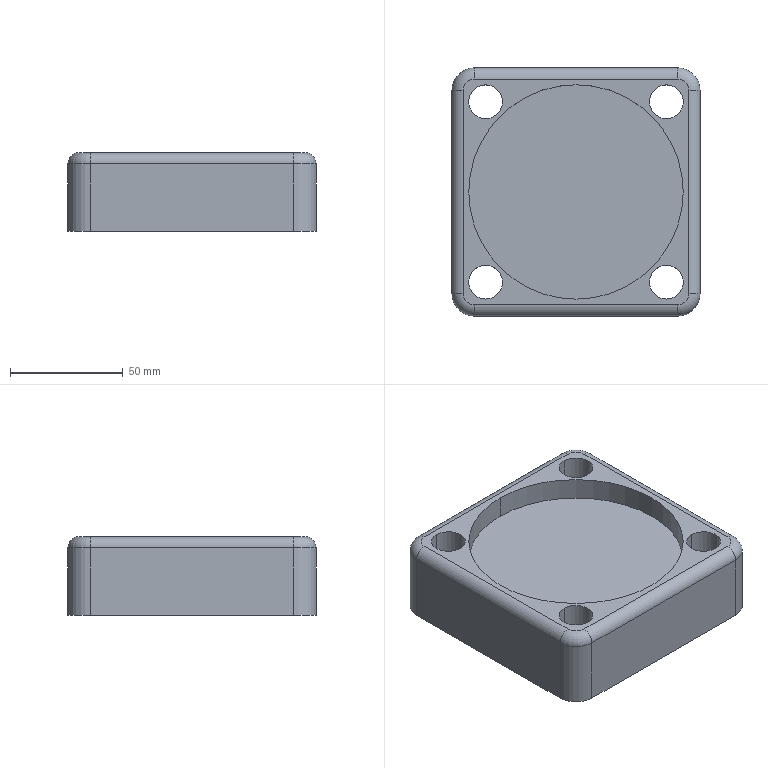Component | SolidWorks | MountingBracket-1 | 1 solid | 29 faces | box 110 x 110 x 35 mm | volume 322642 mm3 | cylinder 18 | plane 7 | torus 4 | commonest cylinder face diameters 15 x8 20 x4 10 x4 95 x2 | material 1023 Carbon Steel Plate (SS)
build123d program:
from build123d import *

# Parameters (mm, degrees)
SKETCH1_W           = 110
SKETCH1_H           = 110
BOSS_EXTRUDE1_DEPTH = 17.5
SKETCH2_R           = 47.5
CUT_EXTRUDE1_DEPTH  = 10
SKETCH3_R           = 7.5
CUT_EXTRUDE2_DEPTH  = 86.294
FILLET1_R           = 10
FILLET2_R           = 5


with BuildPart() as part:
    # Sketch1 → Boss-Extrude1 (new, symmetric)
    with BuildSketch(Plane.XY):
        Rectangle(SKETCH1_W, SKETCH1_H)
    extrude(amount=BOSS_EXTRUDE1_DEPTH, both=True)

    # Sketch2 → Cut-Extrude1 (cut)
    with BuildSketch(Plane.XY.offset(17.5)):
        Circle(SKETCH2_R)
    extrude(amount=-CUT_EXTRUDE1_DEPTH, mode=Mode.SUBTRACT)

    # Sketch3 → Cut-Extrude2 (cut, through all)
    with BuildSketch(Plane.XY.offset(17.5)):
        with Locations((-40, 40)):
            Circle(SKETCH3_R)
        with Locations(Location((40, 40, 0), (0, 0, 180))):
            Circle(SKETCH3_R)
        with Locations((40, -40)):
            Circle(SKETCH3_R)
        with Locations(Location((-40, -40, 0), (0, 0, 180))):
            Circle(SKETCH3_R)
    extrude(amount=-CUT_EXTRUDE2_DEPTH, mode=Mode.SUBTRACT)

    # Fillet1
    fillet1_edges = [part.edges().sort_by_distance(p)[0] for p in [
        (-55, 55, 0),
        (55, 55, 0),
        (55, -55, 0),
        (-55, -55, 0),
    ]]
    fillet(fillet1_edges, radius=FILLET1_R)

    # Fillet2
    fillet2_edges = [part.edges().sort_by_distance(p)[0] for p in [
        (55, 0, 17.5),
        (0, -55, 17.5),
        (-55, 0, 17.5),
        (0, 55, 17.5),
        (52.071, 52.071, 17.5),
        (-52.071, 52.071, 17.5),
        (-52.071, -52.071, 17.5),
        (52.071, -52.071, 17.5),
    ]]
    fillet(fillet2_edges, radius=FILLET2_R)


solid = part.part

# Placed as in the assembly
solid = solid.moved(Location((-7.456, 2.584, -382.5), (0, 0, 0)))
STEP:
#1=COLOUR_RGB('',0.7922,0.8196,0.9333);
#2=FILL_AREA_STYLE_COLOUR('',#1);
#3=FILL_AREA_STYLE('',(#2));
#4=SURFACE_STYLE_FILL_AREA(#3);
#5=SURFACE_SIDE_STYLE('',(#4));
#6=SURFACE_STYLE_USAGE(.BOTH.,#5);
#7=PRESENTATION_STYLE_ASSIGNMENT((#6));
#8=CARTESIAN_POINT('',(-1.868,1.972,-15.748));
#9=VERTEX_POINT('',#8);
#10=CARTESIAN_POINT('',(-1.868,1.381,-15.748));
#11=VERTEX_POINT('',#10);
#12=CARTESIAN_POINT('',(-1.868,1.677,-15.748));
#13=DIRECTION('',(-0.,-0.,1.));
#14=DIRECTION('',(0.,1.,0.));
#15=AXIS2_PLACEMENT_3D('',#12,#13,#14);
#16=CIRCLE('',#15,0.2953);
#17=EDGE_CURVE('',#9,#11,#16,.T.);
#18=ORIENTED_EDGE('',*,*,#17,.F.);
#19=CARTESIAN_POINT('',(-1.868,1.972,-14.37));
#20=VERTEX_POINT('',#19);
#21=CARTESIAN_POINT('',(-1.868,1.972,-15.748));
#22=DIRECTION('',(-0.,-0.,1.));
#23=VECTOR('',#22,39.37);
#24=LINE('',#21,#23);
#25=EDGE_CURVE('',#9,#20,#24,.T.);
#26=ORIENTED_EDGE('',*,*,#25,.T.);
#27=CARTESIAN_POINT('',(-1.868,1.381,-14.37));
#28=VERTEX_POINT('',#27);
#29=CARTESIAN_POINT('',(-1.868,1.677,-14.37));
#30=DIRECTION('',(-0.,-0.,1.));
#31=DIRECTION('',(0.,1.,0.));
#32=AXIS2_PLACEMENT_3D('',#29,#30,#31);
#33=CIRCLE('',#32,0.2953);
#34=EDGE_CURVE('',#20,#28,#33,.T.);
#35=ORIENTED_EDGE('',*,*,#34,.T.);
#36=CARTESIAN_POINT('',(-1.868,1.381,-15.748));
#37=DIRECTION('',(-0.,-0.,1.));
#38=VECTOR('',#37,39.37);
#39=LINE('',#36,#38);
#40=EDGE_CURVE('',#11,#28,#39,.T.);
#41=ORIENTED_EDGE('',*,*,#40,.F.);
#42=EDGE_LOOP('',(#18,#26,#35,#41));
#43=FACE_OUTER_BOUND('',#42,.T.);
#44=CARTESIAN_POINT('',(-1.868,1.677,-15.748));
#45=DIRECTION('',(-0.,-0.,1.));
#46=DIRECTION('',(0.,-1.,0.));
#47=AXIS2_PLACEMENT_3D('',#44,#45,#46);
#48=CYLINDRICAL_SURFACE('',#47,0.2953);
#49=ADVANCED_FACE('',(#43),#48,.F.);
#50=CARTESIAN_POINT('',(-1.868,-1.178,-15.748));
#51=VERTEX_POINT('',#50);
#52=CARTESIAN_POINT('',(-1.868,-1.768,-15.748));
#53=VERTEX_POINT('',#52);
#54=CARTESIAN_POINT('',(-1.868,-1.473,-15.748));
#55=DIRECTION('',(-0.,-0.,1.));
#56=DIRECTION('',(0.,-1.,0.));
#57=AXIS2_PLACEMENT_3D('',#54,#55,#56);
#58=CIRCLE('',#57,0.2953);
#59=EDGE_CURVE('',#51,#53,#58,.T.);
#60=ORIENTED_EDGE('',*,*,#59,.F.);
#61=CARTESIAN_POINT('',(-1.868,-1.178,-14.37));
#62=VERTEX_POINT('',#61);
#63=CARTESIAN_POINT('',(-1.868,-1.178,-15.748));
#64=DIRECTION('',(-0.,-0.,1.));
#65=VECTOR('',#64,39.37);
#66=LINE('',#63,#65);
#67=EDGE_CURVE('',#51,#62,#66,.T.);
#68=ORIENTED_EDGE('',*,*,#67,.T.);
#69=CARTESIAN_POINT('',(-1.868,-1.768,-14.37));
#70=VERTEX_POINT('',#69);
#71=CARTESIAN_POINT('',(-1.868,-1.473,-14.37));
#72=DIRECTION('',(-0.,-0.,1.));
#73=DIRECTION('',(0.,-1.,0.));
#74=AXIS2_PLACEMENT_3D('',#71,#72,#73);
#75=CIRCLE('',#74,0.2953);
#76=EDGE_CURVE('',#62,#70,#75,.T.);
#77=ORIENTED_EDGE('',*,*,#76,.T.);
#78=CARTESIAN_POINT('',(-1.868,-1.768,-15.748));
#79=DIRECTION('',(-0.,-0.,1.));
#80=VECTOR('',#79,39.37);
#81=LINE('',#78,#80);
#82=EDGE_CURVE('',#53,#70,#81,.T.);
#83=ORIENTED_EDGE('',*,*,#82,.F.);
#84=EDGE_LOOP('',(#60,#68,#77,#83));
#85=FACE_OUTER_BOUND('',#84,.T.);
#86=CARTESIAN_POINT('',(-1.868,-1.473,-15.748));
#87=DIRECTION('',(-0.,-0.,1.));
#88=DIRECTION('',(0.,-1.,0.));
#89=AXIS2_PLACEMENT_3D('',#86,#87,#88);
#90=CYLINDRICAL_SURFACE('',#89,0.2953);
#91=ADVANCED_FACE('',(#85),#90,.F.);
#92=CARTESIAN_POINT('',(1.281,-1.178,-15.748));
#93=VERTEX_POINT('',#92);
#94=CARTESIAN_POINT('',(1.281,-1.768,-15.748));
#95=VERTEX_POINT('',#94);
#96=CARTESIAN_POINT('',(1.281,-1.473,-15.748));
#97=DIRECTION('',(-0.,-0.,1.));
#98=DIRECTION('',(0.,1.,0.));
#99=AXIS2_PLACEMENT_3D('',#96,#97,#98);
#100=CIRCLE('',#99,0.2953);
#101=EDGE_CURVE('',#93,#95,#100,.T.);
#102=ORIENTED_EDGE('',*,*,#101,.F.);
#103=CARTESIAN_POINT('',(1.281,-1.178,-14.37));
#104=VERTEX_POINT('',#103);
#105=CARTESIAN_POINT('',(1.281,-1.178,-15.748));
#106=DIRECTION('',(-0.,-0.,1.));
#107=VECTOR('',#106,39.37);
#108=LINE('',#105,#107);
#109=EDGE_CURVE('',#93,#104,#108,.T.);
#110=ORIENTED_EDGE('',*,*,#109,.T.);
#111=CARTESIAN_POINT('',(1.281,-1.768,-14.37));
#112=VERTEX_POINT('',#111);
#113=CARTESIAN_POINT('',(1.281,-1.473,-14.37));
#114=DIRECTION('',(-0.,-0.,1.));
#115=DIRECTION('',(0.,1.,0.));
#116=AXIS2_PLACEMENT_3D('',#113,#114,#115);
#117=CIRCLE('',#116,0.2953);
#118=EDGE_CURVE('',#104,#112,#117,.T.);
#119=ORIENTED_EDGE('',*,*,#118,.T.);
#120=CARTESIAN_POINT('',(1.281,-1.768,-15.748));
#121=DIRECTION('',(-0.,-0.,1.));
#122=VECTOR('',#121,39.37);
#123=LINE('',#120,#122);
#124=EDGE_CURVE('',#95,#112,#123,.T.);
#125=ORIENTED_EDGE('',*,*,#124,.F.);
#126=EDGE_LOOP('',(#102,#110,#119,#125));
#127=FACE_OUTER_BOUND('',#126,.T.);
#128=CARTESIAN_POINT('',(1.281,-1.473,-15.748));
#129=DIRECTION('',(-0.,-0.,1.));
#130=DIRECTION('',(0.,-1.,0.));
#131=AXIS2_PLACEMENT_3D('',#128,#129,#130);
#132=CYLINDRICAL_SURFACE('',#131,0.2953);
#133=ADVANCED_FACE('',(#127),#132,.F.);
#134=CARTESIAN_POINT('',(1.281,1.972,-15.748));
#135=VERTEX_POINT('',#134);
#136=CARTESIAN_POINT('',(1.281,1.381,-15.748));
#137=VERTEX_POINT('',#136);
#138=CARTESIAN_POINT('',(1.281,1.677,-15.748));
#139=DIRECTION('',(-0.,-0.,1.));
#140=DIRECTION('',(0.,-1.,0.));
#141=AXIS2_PLACEMENT_3D('',#138,#139,#140);
#142=CIRCLE('',#141,0.2953);
#143=EDGE_CURVE('',#135,#137,#142,.T.);
#144=ORIENTED_EDGE('',*,*,#143,.F.);
#145=CARTESIAN_POINT('',(1.281,1.972,-14.37));
#146=VERTEX_POINT('',#145);
#147=CARTESIAN_POINT('',(1.281,1.972,-15.748));
#148=DIRECTION('',(-0.,-0.,1.));
#149=VECTOR('',#148,39.37);
#150=LINE('',#147,#149);
#151=EDGE_CURVE('',#135,#146,#150,.T.);
#152=ORIENTED_EDGE('',*,*,#151,.T.);
#153=CARTESIAN_POINT('',(1.281,1.381,-14.37));
#154=VERTEX_POINT('',#153);
#155=CARTESIAN_POINT('',(1.281,1.677,-14.37));
#156=DIRECTION('',(-0.,-0.,1.));
#157=DIRECTION('',(0.,-1.,0.));
#158=AXIS2_PLACEMENT_3D('',#155,#156,#157);
#159=CIRCLE('',#158,0.2953);
#160=EDGE_CURVE('',#146,#154,#159,.T.);
#161=ORIENTED_EDGE('',*,*,#160,.T.);
#162=CARTESIAN_POINT('',(1.281,1.381,-15.748));
#163=DIRECTION('',(-0.,-0.,1.));
#164=VECTOR('',#163,39.37);
#165=LINE('',#162,#164);
#166=EDGE_CURVE('',#137,#154,#165,.T.);
#167=ORIENTED_EDGE('',*,*,#166,.F.);
#168=EDGE_LOOP('',(#144,#152,#161,#167));
#169=FACE_OUTER_BOUND('',#168,.T.);
#170=CARTESIAN_POINT('',(1.281,1.677,-15.748));
#171=DIRECTION('',(-0.,-0.,1.));
#172=DIRECTION('',(0.,-1.,0.));
#173=AXIS2_PLACEMENT_3D('',#170,#171,#172);
#174=CYLINDRICAL_SURFACE('',#173,0.2953);
#175=ADVANCED_FACE('',(#169),#174,.F.);
#176=CARTESIAN_POINT('',(-0.2935,1.972,-14.764));
#177=VERTEX_POINT('',#176);
#178=CARTESIAN_POINT('',(-0.2935,-1.768,-14.764));
#179=VERTEX_POINT('',#178);
#180=CARTESIAN_POINT('',(-0.2935,0.1017,-14.764));
#181=DIRECTION('',(-0.,-0.,1.));
#182=DIRECTION('',(-0.,-1.,0.));
#183=AXIS2_PLACEMENT_3D('',#180,#181,#182);
#184=CIRCLE('',#183,1.87);
#185=EDGE_CURVE('',#177,#179,#184,.T.);
#186=ORIENTED_EDGE('',*,*,#185,.F.);
#187=CARTESIAN_POINT('',(-0.2935,1.972,-14.37));
#188=VERTEX_POINT('',#187);
#189=CARTESIAN_POINT('',(-0.2935,1.972,-14.764));
#190=DIRECTION('',(-0.,-0.,1.));
#191=VECTOR('',#190,39.37);
#192=LINE('',#189,#191);
#193=EDGE_CURVE('',#177,#188,#192,.T.);
#194=ORIENTED_EDGE('',*,*,#193,.T.);
#195=CARTESIAN_POINT('',(-0.2935,-1.768,-14.37));
#196=VERTEX_POINT('',#195);
#197=CARTESIAN_POINT('',(-0.2935,0.1017,-14.37));
#198=DIRECTION('',(-0.,-0.,1.));
#199=DIRECTION('',(-0.,-1.,0.));
#200=AXIS2_PLACEMENT_3D('',#197,#198,#199);
#201=CIRCLE('',#200,1.87);
#202=EDGE_CURVE('',#188,#196,#201,.T.);
#203=ORIENTED_EDGE('',*,*,#202,.T.);
#204=CARTESIAN_POINT('',(-0.2935,-1.768,-14.764));
#205=DIRECTION('',(-0.,-0.,1.));
#206=VECTOR('',#205,39.37);
#207=LINE('',#204,#206);
#208=EDGE_CURVE('',#179,#196,#207,.T.);
#209=ORIENTED_EDGE('',*,*,#208,.F.);
#210=EDGE_LOOP('',(#186,#194,#203,#209));
#211=FACE_OUTER_BOUND('',#210,.T.);
#212=CARTESIAN_POINT('',(-0.2935,0.1017,-14.764));
#213=DIRECTION('',(-0.,-0.,1.));
#214=DIRECTION('',(-0.,-1.,0.));
#215=AXIS2_PLACEMENT_3D('',#212,#213,#214);
#216=CYLINDRICAL_SURFACE('',#215,1.87);
#217=ADVANCED_FACE('',(#211),#216,.F.);
#218=CARTESIAN_POINT('',(-2.065,2.267,-15.748));
#219=VERTEX_POINT('',#218);
#220=CARTESIAN_POINT('',(-2.065,2.267,-14.567));
#221=VERTEX_POINT('',#220);
#222=CARTESIAN_POINT('',(-2.065,2.267,-14.37));
#223=DIRECTION('',(-0.,-0.,1.));
#224=VECTOR('',#223,39.37);
#225=LINE('',#222,#224);
#226=EDGE_CURVE('',#219,#221,#225,.T.);
#227=ORIENTED_EDGE('',*,*,#226,.T.);
#228=CARTESIAN_POINT('',(1.478,2.267,-14.567));
#229=VERTEX_POINT('',#228);
#230=CARTESIAN_POINT('',(1.478,2.267,-14.567));
#231=DIRECTION('',(1.,-0.,0.));
#232=VECTOR('',#231,39.37);
#233=LINE('',#230,#232);
#234=EDGE_CURVE('',#221,#229,#233,.T.);
#235=ORIENTED_EDGE('',*,*,#234,.T.);
#236=CARTESIAN_POINT('',(1.478,2.267,-15.748));
#237=VERTEX_POINT('',#236);
#238=CARTESIAN_POINT('',(1.478,2.267,-14.37));
#239=DIRECTION('',(0.,0.,-1.));
#240=VECTOR('',#239,39.37);
#241=LINE('',#238,#240);
#242=EDGE_CURVE('',#229,#237,#241,.T.);
#243=ORIENTED_EDGE('',*,*,#242,.T.);
#244=CARTESIAN_POINT('',(-2.459,2.267,-15.748));
#245=DIRECTION('',(-1.,0.,-0.));
#246=VECTOR('',#245,39.37);
#247=LINE('',#244,#246);
#248=EDGE_CURVE('',#237,#219,#247,.T.);
#249=ORIENTED_EDGE('',*,*,#248,.T.);
#250=EDGE_LOOP('',(#227,#235,#243,#249));
#251=FACE_OUTER_BOUND('',#250,.T.);
#252=CARTESIAN_POINT('',(-2.459,2.267,-14.37));
#253=DIRECTION('',(-0.,-1.,-0.));
#254=DIRECTION('',(0.,0.,-1.));
#255=AXIS2_PLACEMENT_3D('',#252,#253,#254);
#256=PLANE('',#255);
#257=ADVANCED_FACE('',(#251),#256,.F.);
#258=CARTESIAN_POINT('',(-2.459,-1.67,-15.748));
#259=VERTEX_POINT('',#258);
#260=CARTESIAN_POINT('',(-2.459,-1.67,-14.567));
#261=VERTEX_POINT('',#260);
#262=CARTESIAN_POINT('',(-2.459,-1.67,-14.37));
#263=DIRECTION('',(-0.,-0.,1.));
#264=VECTOR('',#263,39.37);
#265=LINE('',#262,#264);
#266=EDGE_CURVE('',#259,#261,#265,.T.);
#267=ORIENTED_EDGE('',*,*,#266,.T.);
#268=CARTESIAN_POINT('',(-2.459,1.873,-14.567));
#269=VERTEX_POINT('',#268);
#270=CARTESIAN_POINT('',(-2.459,1.873,-14.567));
#271=DIRECTION('',(0.,1.,0.));
#272=VECTOR('',#271,39.37);
#273=LINE('',#270,#272);
#274=EDGE_CURVE('',#261,#269,#273,.T.);
#275=ORIENTED_EDGE('',*,*,#274,.T.);
#276=CARTESIAN_POINT('',(-2.459,1.873,-15.748));
#277=VERTEX_POINT('',#276);
#278=CARTESIAN_POINT('',(-2.459,1.873,-14.37));
#279=DIRECTION('',(0.,0.,-1.));
#280=VECTOR('',#279,39.37);
#281=LINE('',#278,#280);
#282=EDGE_CURVE('',#269,#277,#281,.T.);
#283=ORIENTED_EDGE('',*,*,#282,.T.);
#284=CARTESIAN_POINT('',(-2.459,-2.064,-15.748));
#285=DIRECTION('',(-0.,-1.,-0.));
#286=VECTOR('',#285,39.37);
#287=LINE('',#284,#286);
#288=EDGE_CURVE('',#277,#259,#287,.T.);
#289=ORIENTED_EDGE('',*,*,#288,.T.);
#290=EDGE_LOOP('',(#267,#275,#283,#289));
#291=FACE_OUTER_BOUND('',#290,.T.);
#292=CARTESIAN_POINT('',(-2.459,-2.064,-14.37));
#293=DIRECTION('',(1.,-0.,0.));
#294=DIRECTION('',(0.,1.,0.));
#295=AXIS2_PLACEMENT_3D('',#292,#293,#294);
#296=PLANE('',#295);
#297=ADVANCED_FACE('',(#291),#296,.F.);
#298=CARTESIAN_POINT('',(1.478,-2.064,-15.748));
#299=VERTEX_POINT('',#298);
#300=CARTESIAN_POINT('',(1.478,-2.064,-14.567));
#301=VERTEX_POINT('',#300);
#302=CARTESIAN_POINT('',(1.478,-2.064,-14.37));
#303=DIRECTION('',(-0.,-0.,1.));
#304=VECTOR('',#303,39.37);
#305=LINE('',#302,#304);
#306=EDGE_CURVE('',#299,#301,#305,.T.);
#307=ORIENTED_EDGE('',*,*,#306,.T.);
#308=CARTESIAN_POINT('',(-2.065,-2.064,-14.567));
#309=VERTEX_POINT('',#308);
#310=CARTESIAN_POINT('',(-2.065,-2.064,-14.567));
#311=DIRECTION('',(-1.,0.,-0.));
#312=VECTOR('',#311,39.37);
#313=LINE('',#310,#312);
#314=EDGE_CURVE('',#301,#309,#313,.T.);
#315=ORIENTED_EDGE('',*,*,#314,.T.);
#316=CARTESIAN_POINT('',(-2.065,-2.064,-15.748));
#317=VERTEX_POINT('',#316);
#318=CARTESIAN_POINT('',(-2.065,-2.064,-14.37));
#319=DIRECTION('',(0.,0.,-1.));
#320=VECTOR('',#319,39.37);
#321=LINE('',#318,#320);
#322=EDGE_CURVE('',#309,#317,#321,.T.);
#323=ORIENTED_EDGE('',*,*,#322,.T.);
#324=CARTESIAN_POINT('',(-2.459,-2.064,-15.748));
#325=DIRECTION('',(1.,-0.,0.));
#326=VECTOR('',#325,39.37);
#327=LINE('',#324,#326);
#328=EDGE_CURVE('',#317,#299,#327,.T.);
#329=ORIENTED_EDGE('',*,*,#328,.T.);
#330=EDGE_LOOP('',(#307,#315,#323,#329));
#331=FACE_OUTER_BOUND('',#330,.T.);
#332=CARTESIAN_POINT('',(-2.459,-2.064,-14.37));
#333=DIRECTION('',(0.,1.,0.));
#334=DIRECTION('',(-0.,-0.,1.));
#335=AXIS2_PLACEMENT_3D('',#332,#333,#334);
#336=PLANE('',#335);
#337=ADVANCED_FACE('',(#331),#336,.F.);
#338=CARTESIAN_POINT('',(1.872,1.873,-15.748));
#339=VERTEX_POINT('',#338);
#340=CARTESIAN_POINT('',(1.872,1.873,-14.567));
#341=VERTEX_POINT('',#340);
#342=CARTESIAN_POINT('',(1.872,1.873,-14.37));
#343=DIRECTION('',(-0.,-0.,1.));
#344=VECTOR('',#343,39.37);
#345=LINE('',#342,#344);
#346=EDGE_CURVE('',#339,#341,#345,.T.);
#347=ORIENTED_EDGE('',*,*,#346,.T.);
#348=CARTESIAN_POINT('',(1.872,-1.67,-14.567));
#349=VERTEX_POINT('',#348);
#350=CARTESIAN_POINT('',(1.872,-1.67,-14.567));
#351=DIRECTION('',(-0.,-1.,-0.));
#352=VECTOR('',#351,39.37);
#353=LINE('',#350,#352);
#354=EDGE_CURVE('',#341,#349,#353,.T.);
#355=ORIENTED_EDGE('',*,*,#354,.T.);
#356=CARTESIAN_POINT('',(1.872,-1.67,-15.748));
#357=VERTEX_POINT('',#356);
#358=CARTESIAN_POINT('',(1.872,-1.67,-14.37));
#359=DIRECTION('',(0.,0.,-1.));
#360=VECTOR('',#359,39.37);
#361=LINE('',#358,#360);
#362=EDGE_CURVE('',#349,#357,#361,.T.);
#363=ORIENTED_EDGE('',*,*,#362,.T.);
#364=CARTESIAN_POINT('',(1.872,-2.064,-15.748));
#365=DIRECTION('',(0.,1.,0.));
#366=VECTOR('',#365,39.37);
#367=LINE('',#364,#366);
#368=EDGE_CURVE('',#357,#339,#367,.T.);
#369=ORIENTED_EDGE('',*,*,#368,.T.);
#370=EDGE_LOOP('',(#347,#355,#363,#369));
#371=FACE_OUTER_BOUND('',#370,.T.);
#372=CARTESIAN_POINT('',(1.872,-2.064,-14.37));
#373=DIRECTION('',(-1.,0.,-0.));
#374=DIRECTION('',(-0.,-1.,-0.));
#375=AXIS2_PLACEMENT_3D('',#372,#373,#374);
#376=PLANE('',#375);
#377=ADVANCED_FACE('',(#371),#376,.F.);
#378=CARTESIAN_POINT('',(-2.065,2.07,-14.37));
#379=VERTEX_POINT('',#378);
#380=CARTESIAN_POINT('',(-2.262,1.873,-14.37));
#381=VERTEX_POINT('',#380);
#382=CARTESIAN_POINT('',(-2.065,1.873,-14.37));
#383=DIRECTION('',(-0.,-0.,1.));
#384=DIRECTION('',(0.,-1.,0.));
#385=AXIS2_PLACEMENT_3D('',#382,#383,#384);
#386=CIRCLE('',#385,0.1969);
#387=EDGE_CURVE('',#379,#381,#386,.T.);
#388=ORIENTED_EDGE('',*,*,#387,.T.);
#389=CARTESIAN_POINT('',(-2.262,-1.67,-14.37));
#390=VERTEX_POINT('',#389);
#391=CARTESIAN_POINT('',(-2.262,-1.67,-14.37));
#392=DIRECTION('',(-0.,-1.,-0.));
#393=VECTOR('',#392,39.37);
#394=LINE('',#391,#393);
#395=EDGE_CURVE('',#381,#390,#394,.T.);
#396=ORIENTED_EDGE('',*,*,#395,.T.);
#397=CARTESIAN_POINT('',(-2.065,-1.867,-14.37));
#398=VERTEX_POINT('',#397);
#399=CARTESIAN_POINT('',(-2.065,-1.67,-14.37));
#400=DIRECTION('',(-0.,-0.,1.));
#401=DIRECTION('',(0.,-1.,0.));
#402=AXIS2_PLACEMENT_3D('',#399,#400,#401);
#403=CIRCLE('',#402,0.1969);
#404=EDGE_CURVE('',#390,#398,#403,.T.);
#405=ORIENTED_EDGE('',*,*,#404,.T.);
#406=CARTESIAN_POINT('',(1.478,-1.867,-14.37));
#407=VERTEX_POINT('',#406);
#408=CARTESIAN_POINT('',(1.478,-1.867,-14.37));
#409=DIRECTION('',(1.,-0.,0.));
#410=VECTOR('',#409,39.37);
#411=LINE('',#408,#410);
#412=EDGE_CURVE('',#398,#407,#411,.T.);
#413=ORIENTED_EDGE('',*,*,#412,.T.);
#414=CARTESIAN_POINT('',(1.675,-1.67,-14.37));
#415=VERTEX_POINT('',#414);
#416=CARTESIAN_POINT('',(1.478,-1.67,-14.37));
#417=DIRECTION('',(-0.,-0.,1.));
#418=DIRECTION('',(0.,-1.,0.));
#419=AXIS2_PLACEMENT_3D('',#416,#417,#418);
#420=CIRCLE('',#419,0.1969);
#421=EDGE_CURVE('',#407,#415,#420,.T.);
#422=ORIENTED_EDGE('',*,*,#421,.T.);
#423=CARTESIAN_POINT('',(1.675,1.873,-14.37));
#424=VERTEX_POINT('',#423);
#425=CARTESIAN_POINT('',(1.675,1.873,-14.37));
#426=DIRECTION('',(0.,1.,0.));
#427=VECTOR('',#426,39.37);
#428=LINE('',#425,#427);
#429=EDGE_CURVE('',#415,#424,#428,.T.);
#430=ORIENTED_EDGE('',*,*,#429,.T.);
#431=CARTESIAN_POINT('',(1.478,2.07,-14.37));
#432=VERTEX_POINT('',#431);
#433=CARTESIAN_POINT('',(1.478,1.873,-14.37));
#434=DIRECTION('',(-0.,-0.,1.));
#435=DIRECTION('',(0.,-1.,0.));
#436=AXIS2_PLACEMENT_3D('',#433,#434,#435);
#437=CIRCLE('',#436,0.1969);
#438=EDGE_CURVE('',#424,#432,#437,.T.);
#439=ORIENTED_EDGE('',*,*,#438,.T.);
#440=CARTESIAN_POINT('',(-2.065,2.07,-14.37));
#441=DIRECTION('',(-1.,0.,-0.));
#442=VECTOR('',#441,39.37);
#443=LINE('',#440,#442);
#444=EDGE_CURVE('',#432,#379,#443,.T.);
#445=ORIENTED_EDGE('',*,*,#444,.T.);
#446=EDGE_LOOP('',(#388,#396,#405,#413,#422,#430,#439,#445));
#447=FACE_OUTER_BOUND('',#446,.T.);
#448=CARTESIAN_POINT('',(-1.868,1.677,-14.37));
#449=DIRECTION('',(-0.,-0.,1.));
#450=DIRECTION('',(0.,1.,0.));
#451=AXIS2_PLACEMENT_3D('',#448,#449,#450);
#452=CIRCLE('',#451,0.2953);
#453=EDGE_CURVE('',#28,#20,#452,.T.);
#454=ORIENTED_EDGE('',*,*,#453,.F.);
#455=ORIENTED_EDGE('',*,*,#34,.F.);
#456=EDGE_LOOP('',(#454,#455));
#457=FACE_BOUND('',#456,.T.);
#458=CARTESIAN_POINT('',(-1.868,-1.473,-14.37));
#459=DIRECTION('',(-0.,-0.,1.));
#460=DIRECTION('',(0.,-1.,0.));
#461=AXIS2_PLACEMENT_3D('',#458,#459,#460);
#462=CIRCLE('',#461,0.2953);
#463=EDGE_CURVE('',#70,#62,#462,.T.);
#464=ORIENTED_EDGE('',*,*,#463,.F.);
#465=ORIENTED_EDGE('',*,*,#76,.F.);
#466=EDGE_LOOP('',(#464,#465));
#467=FACE_BOUND('',#466,.T.);
#468=CARTESIAN_POINT('',(1.281,-1.473,-14.37));
#469=DIRECTION('',(-0.,-0.,1.));
#470=DIRECTION('',(0.,1.,0.));
#471=AXIS2_PLACEMENT_3D('',#468,#469,#470);
#472=CIRCLE('',#471,0.2953);
#473=EDGE_CURVE('',#112,#104,#472,.T.);
#474=ORIENTED_EDGE('',*,*,#473,.F.);
#475=ORIENTED_EDGE('',*,*,#118,.F.);
#476=EDGE_LOOP('',(#474,#475));
#477=FACE_BOUND('',#476,.T.);
#478=CARTESIAN_POINT('',(1.281,1.677,-14.37));
#479=DIRECTION('',(-0.,-0.,1.));
#480=DIRECTION('',(0.,-1.,0.));
#481=AXIS2_PLACEMENT_3D('',#478,#479,#480);
#482=CIRCLE('',#481,0.2953);
#483=EDGE_CURVE('',#154,#146,#482,.T.);
#484=ORIENTED_EDGE('',*,*,#483,.F.);
#485=ORIENTED_EDGE('',*,*,#160,.F.);
#486=EDGE_LOOP('',(#484,#485));
#487=FACE_BOUND('',#486,.T.);
#488=CARTESIAN_POINT('',(-0.2935,0.1017,-14.37));
#489=DIRECTION('',(-0.,-0.,1.));
#490=DIRECTION('',(-0.,-1.,0.));
#491=AXIS2_PLACEMENT_3D('',#488,#489,#490);
#492=CIRCLE('',#491,1.87);
#493=EDGE_CURVE('',#196,#188,#492,.T.);
#494=ORIENTED_EDGE('',*,*,#493,.F.);
#495=ORIENTED_EDGE('',*,*,#202,.F.);
#496=EDGE_LOOP('',(#494,#495));
#497=FACE_BOUND('',#496,.T.);
#498=CARTESIAN_POINT('',(1.872,2.267,-14.37));
#499=DIRECTION('',(-0.,-0.,1.));
#500=DIRECTION('',(-0.,-1.,-0.));
#501=AXIS2_PLACEMENT_3D('',#498,#499,#500);
#502=PLANE('',#501);
#503=ADVANCED_FACE('',(#447,#457,#467,#477,#487,#497),#502,.T.);
#504=CARTESIAN_POINT('',(-1.868,1.677,-15.748));
#505=DIRECTION('',(-0.,-0.,1.));
#506=DIRECTION('',(0.,1.,0.));
#507=AXIS2_PLACEMENT_3D('',#504,#505,#506);
#508=CIRCLE('',#507,0.2953);
#509=EDGE_CURVE('',#11,#9,#508,.T.);
#510=ORIENTED_EDGE('',*,*,#509,.T.);
#511=ORIENTED_EDGE('',*,*,#17,.T.);
#512=EDGE_LOOP('',(#510,#511));
#513=FACE_BOUND('',#512,.T.);
#514=CARTESIAN_POINT('',(-1.868,-1.473,-15.748));
#515=DIRECTION('',(-0.,-0.,1.));
#516=DIRECTION('',(0.,-1.,0.));
#517=AXIS2_PLACEMENT_3D('',#514,#515,#516);
#518=CIRCLE('',#517,0.2953);
#519=EDGE_CURVE('',#53,#51,#518,.T.);
#520=ORIENTED_EDGE('',*,*,#519,.T.);
#521=ORIENTED_EDGE('',*,*,#59,.T.);
#522=EDGE_LOOP('',(#520,#521));
#523=FACE_BOUND('',#522,.T.);
#524=CARTESIAN_POINT('',(1.281,-1.473,-15.748));
#525=DIRECTION('',(-0.,-0.,1.));
#526=DIRECTION('',(0.,1.,0.));
#527=AXIS2_PLACEMENT_3D('',#524,#525,#526);
#528=CIRCLE('',#527,0.2953);
#529=EDGE_CURVE('',#95,#93,#528,.T.);
#530=ORIENTED_EDGE('',*,*,#529,.T.);
#531=ORIENTED_EDGE('',*,*,#101,.T.);
#532=EDGE_LOOP('',(#530,#531));
#533=FACE_BOUND('',#532,.T.);
#534=CARTESIAN_POINT('',(1.281,1.677,-15.748));
#535=DIRECTION('',(-0.,-0.,1.));
#536=DIRECTION('',(0.,-1.,0.));
#537=AXIS2_PLACEMENT_3D('',#534,#535,#536);
#538=CIRCLE('',#537,0.2953);
#539=EDGE_CURVE('',#137,#135,#538,.T.);
#540=ORIENTED_EDGE('',*,*,#539,.T.);
#541=ORIENTED_EDGE('',*,*,#143,.T.);
#542=EDGE_LOOP('',(#540,#541));
#543=FACE_BOUND('',#542,.T.);
#544=ORIENTED_EDGE('',*,*,#328,.F.);
#545=CARTESIAN_POINT('',(-2.065,-1.67,-15.748));
#546=DIRECTION('',(0.,0.,-1.));
#547=DIRECTION('',(-0.,-1.,0.));
#548=AXIS2_PLACEMENT_3D('',#545,#546,#547);
#549=CIRCLE('',#548,0.3937);
#550=EDGE_CURVE('',#317,#259,#549,.T.);
#551=ORIENTED_EDGE('',*,*,#550,.T.);
#552=ORIENTED_EDGE('',*,*,#288,.F.);
#553=CARTESIAN_POINT('',(-2.065,1.873,-15.748));
#554=DIRECTION('',(0.,0.,-1.));
#555=DIRECTION('',(0.,-1.,0.));
#556=AXIS2_PLACEMENT_3D('',#553,#554,#555);
#557=CIRCLE('',#556,0.3937);
#558=EDGE_CURVE('',#277,#219,#557,.T.);
#559=ORIENTED_EDGE('',*,*,#558,.T.);
#560=ORIENTED_EDGE('',*,*,#248,.F.);
#561=CARTESIAN_POINT('',(1.478,1.873,-15.748));
#562=DIRECTION('',(0.,0.,-1.));
#563=DIRECTION('',(0.,-1.,0.));
#564=AXIS2_PLACEMENT_3D('',#561,#562,#563);
#565=CIRCLE('',#564,0.3937);
#566=EDGE_CURVE('',#237,#339,#565,.T.);
#567=ORIENTED_EDGE('',*,*,#566,.T.);
#568=ORIENTED_EDGE('',*,*,#368,.F.);
#569=CARTESIAN_POINT('',(1.478,-1.67,-15.748));
#570=DIRECTION('',(0.,0.,-1.));
#571=DIRECTION('',(-0.,-1.,0.));
#572=AXIS2_PLACEMENT_3D('',#569,#570,#571);
#573=CIRCLE('',#572,0.3937);
#574=EDGE_CURVE('',#357,#299,#573,.T.);
#575=ORIENTED_EDGE('',*,*,#574,.T.);
#576=EDGE_LOOP('',(#544,#551,#552,#559,#560,#567,#568,#575));
#577=FACE_OUTER_BOUND('',#576,.T.);
#578=CARTESIAN_POINT('',(1.872,2.267,-15.748));
#579=DIRECTION('',(-0.,-0.,1.));
#580=DIRECTION('',(-0.,-1.,-0.));
#581=AXIS2_PLACEMENT_3D('',#578,#579,#580);
#582=PLANE('',#581);
#583=ADVANCED_FACE('',(#513,#523,#533,#543,#577),#582,.F.);
#584=ORIENTED_EDGE('',*,*,#193,.F.);
#585=CARTESIAN_POINT('',(-0.2935,0.1017,-14.764));
#586=DIRECTION('',(-0.,-0.,1.));
#587=DIRECTION('',(-0.,-1.,0.));
#588=AXIS2_PLACEMENT_3D('',#585,#586,#587);
#589=CIRCLE('',#588,1.87);
#590=EDGE_CURVE('',#179,#177,#589,.T.);
#591=ORIENTED_EDGE('',*,*,#590,.F.);
#592=ORIENTED_EDGE('',*,*,#208,.T.);
#593=ORIENTED_EDGE('',*,*,#493,.T.);
#594=EDGE_LOOP('',(#584,#591,#592,#593));
#595=FACE_OUTER_BOUND('',#594,.T.);
#596=CARTESIAN_POINT('',(-0.2935,0.1017,-14.764));
#597=DIRECTION('',(-0.,-0.,1.));
#598=DIRECTION('',(-0.,-1.,0.));
#599=AXIS2_PLACEMENT_3D('',#596,#597,#598);
#600=CYLINDRICAL_SURFACE('',#599,1.87);
#601=ADVANCED_FACE('',(#595),#600,.F.);
#602=ORIENTED_EDGE('',*,*,#590,.T.);
#603=ORIENTED_EDGE('',*,*,#185,.T.);
#604=EDGE_LOOP('',(#602,#603));
#605=FACE_OUTER_BOUND('',#604,.T.);
#606=CARTESIAN_POINT('',(-0.2935,0.1017,-14.764));
#607=DIRECTION('',(-0.,-0.,1.));
#608=DIRECTION('',(-0.,-1.,-0.));
#609=AXIS2_PLACEMENT_3D('',#606,#607,#608);
#610=PLANE('',#609);
#611=ADVANCED_FACE('',(#605),#610,.T.);
#612=ORIENTED_EDGE('',*,*,#151,.F.);
#613=ORIENTED_EDGE('',*,*,#539,.F.);
#614=ORIENTED_EDGE('',*,*,#166,.T.);
#615=ORIENTED_EDGE('',*,*,#483,.T.);
#616=EDGE_LOOP('',(#612,#613,#614,#615));
#617=FACE_OUTER_BOUND('',#616,.T.);
#618=CARTESIAN_POINT('',(1.281,1.677,-15.748));
#619=DIRECTION('',(-0.,-0.,1.));
#620=DIRECTION('',(0.,-1.,0.));
#621=AXIS2_PLACEMENT_3D('',#618,#619,#620);
#622=CYLINDRICAL_SURFACE('',#621,0.2953);
#623=ADVANCED_FACE('',(#617),#622,.F.);
#624=ORIENTED_EDGE('',*,*,#109,.F.);
#625=ORIENTED_EDGE('',*,*,#529,.F.);
#626=ORIENTED_EDGE('',*,*,#124,.T.);
#627=ORIENTED_EDGE('',*,*,#473,.T.);
#628=EDGE_LOOP('',(#624,#625,#626,#627));
#629=FACE_OUTER_BOUND('',#628,.T.);
#630=CARTESIAN_POINT('',(1.281,-1.473,-15.748));
#631=DIRECTION('',(-0.,-0.,1.));
#632=DIRECTION('',(0.,-1.,0.));
#633=AXIS2_PLACEMENT_3D('',#630,#631,#632);
#634=CYLINDRICAL_SURFACE('',#633,0.2953);
#635=ADVANCED_FACE('',(#629),#634,.F.);
#636=ORIENTED_EDGE('',*,*,#67,.F.);
#637=ORIENTED_EDGE('',*,*,#519,.F.);
#638=ORIENTED_EDGE('',*,*,#82,.T.);
#639=ORIENTED_EDGE('',*,*,#463,.T.);
#640=EDGE_LOOP('',(#636,#637,#638,#639));
#641=FACE_OUTER_BOUND('',#640,.T.);
#642=CARTESIAN_POINT('',(-1.868,-1.473,-15.748));
#643=DIRECTION('',(-0.,-0.,1.));
#644=DIRECTION('',(0.,-1.,0.));
#645=AXIS2_PLACEMENT_3D('',#642,#643,#644);
#646=CYLINDRICAL_SURFACE('',#645,0.2953);
#647=ADVANCED_FACE('',(#641),#646,.F.);
#648=ORIENTED_EDGE('',*,*,#25,.F.);
#649=ORIENTED_EDGE('',*,*,#509,.F.);
#650=ORIENTED_EDGE('',*,*,#40,.T.);
#651=ORIENTED_EDGE('',*,*,#453,.T.);
#652=EDGE_LOOP('',(#648,#649,#650,#651));
#653=FACE_OUTER_BOUND('',#652,.T.);
#654=CARTESIAN_POINT('',(-1.868,1.677,-15.748));
#655=DIRECTION('',(-0.,-0.,1.));
#656=DIRECTION('',(0.,-1.,0.));
#657=AXIS2_PLACEMENT_3D('',#654,#655,#656);
#658=CYLINDRICAL_SURFACE('',#657,0.2953);
#659=ADVANCED_FACE('',(#653),#658,.F.);
#660=ORIENTED_EDGE('',*,*,#322,.F.);
#661=CARTESIAN_POINT('',(-2.065,-1.67,-14.567));
#662=DIRECTION('',(0.,0.,-1.));
#663=DIRECTION('',(-0.,-1.,0.));
#664=AXIS2_PLACEMENT_3D('',#661,#662,#663);
#665=CIRCLE('',#664,0.3937);
#666=EDGE_CURVE('',#309,#261,#665,.T.);
#667=ORIENTED_EDGE('',*,*,#666,.T.);
#668=ORIENTED_EDGE('',*,*,#266,.F.);
#669=ORIENTED_EDGE('',*,*,#550,.F.);
#670=EDGE_LOOP('',(#660,#667,#668,#669));
#671=FACE_OUTER_BOUND('',#670,.T.);
#672=CARTESIAN_POINT('',(-2.065,-1.67,-14.37));
#673=DIRECTION('',(0.,0.,-1.));
#674=DIRECTION('',(0.,1.,0.));
#675=AXIS2_PLACEMENT_3D('',#672,#673,#674);
#676=CYLINDRICAL_SURFACE('',#675,0.3937);
#677=ADVANCED_FACE('',(#671),#676,.T.);
#678=ORIENTED_EDGE('',*,*,#282,.F.);
#679=CARTESIAN_POINT('',(-2.065,1.873,-14.567));
#680=DIRECTION('',(0.,0.,-1.));
#681=DIRECTION('',(0.,-1.,0.));
#682=AXIS2_PLACEMENT_3D('',#679,#680,#681);
#683=CIRCLE('',#682,0.3937);
#684=EDGE_CURVE('',#269,#221,#683,.T.);
#685=ORIENTED_EDGE('',*,*,#684,.T.);
#686=ORIENTED_EDGE('',*,*,#226,.F.);
#687=ORIENTED_EDGE('',*,*,#558,.F.);
#688=EDGE_LOOP('',(#678,#685,#686,#687));
#689=FACE_OUTER_BOUND('',#688,.T.);
#690=CARTESIAN_POINT('',(-2.065,1.873,-14.37));
#691=DIRECTION('',(0.,0.,-1.));
#692=DIRECTION('',(0.,1.,0.));
#693=AXIS2_PLACEMENT_3D('',#690,#691,#692);
#694=CYLINDRICAL_SURFACE('',#693,0.3937);
#695=ADVANCED_FACE('',(#689),#694,.T.);
#696=ORIENTED_EDGE('',*,*,#242,.F.);
#697=CARTESIAN_POINT('',(1.478,1.873,-14.567));
#698=DIRECTION('',(0.,0.,-1.));
#699=DIRECTION('',(0.,-1.,0.));
#700=AXIS2_PLACEMENT_3D('',#697,#698,#699);
#701=CIRCLE('',#700,0.3937);
#702=EDGE_CURVE('',#229,#341,#701,.T.);
#703=ORIENTED_EDGE('',*,*,#702,.T.);
#704=ORIENTED_EDGE('',*,*,#346,.F.);
#705=ORIENTED_EDGE('',*,*,#566,.F.);
#706=EDGE_LOOP('',(#696,#703,#704,#705));
#707=FACE_OUTER_BOUND('',#706,.T.);
#708=CARTESIAN_POINT('',(1.478,1.873,-14.37));
#709=DIRECTION('',(0.,0.,-1.));
#710=DIRECTION('',(0.,1.,0.));
#711=AXIS2_PLACEMENT_3D('',#708,#709,#710);
#712=CYLINDRICAL_SURFACE('',#711,0.3937);
#713=ADVANCED_FACE('',(#707),#712,.T.);
#714=ORIENTED_EDGE('',*,*,#362,.F.);
#715=CARTESIAN_POINT('',(1.478,-1.67,-14.567));
#716=DIRECTION('',(0.,0.,-1.));
#717=DIRECTION('',(-0.,-1.,0.));
#718=AXIS2_PLACEMENT_3D('',#715,#716,#717);
#719=CIRCLE('',#718,0.3937);
#720=EDGE_CURVE('',#349,#301,#719,.T.);
#721=ORIENTED_EDGE('',*,*,#720,.T.);
#722=ORIENTED_EDGE('',*,*,#306,.F.);
#723=ORIENTED_EDGE('',*,*,#574,.F.);
#724=EDGE_LOOP('',(#714,#721,#722,#723));
#725=FACE_OUTER_BOUND('',#724,.T.);
#726=CARTESIAN_POINT('',(1.478,-1.67,-14.37));
#727=DIRECTION('',(0.,0.,-1.));
#728=DIRECTION('',(0.,1.,0.));
#729=AXIS2_PLACEMENT_3D('',#726,#727,#728);
#730=CYLINDRICAL_SURFACE('',#729,0.3937);
#731=ADVANCED_FACE('',(#725),#730,.T.);
#732=CARTESIAN_POINT('',(-2.065,2.07,-14.567));
#733=DIRECTION('',(1.,-0.,0.));
#734=DIRECTION('',(0.,0.,1.));
#735=AXIS2_PLACEMENT_3D('',#732,#733,#734);
#736=CIRCLE('',#735,0.1969);
#737=EDGE_CURVE('',#221,#379,#736,.T.);
#738=ORIENTED_EDGE('',*,*,#737,.F.);
#739=ORIENTED_EDGE('',*,*,#684,.F.);
#740=CARTESIAN_POINT('',(-2.262,1.873,-14.567));
#741=DIRECTION('',(-0.,-1.,-0.));
#742=DIRECTION('',(0.,0.,-1.));
#743=AXIS2_PLACEMENT_3D('',#740,#741,#742);
#744=CIRCLE('',#743,0.1969);
#745=EDGE_CURVE('',#381,#269,#744,.T.);
#746=ORIENTED_EDGE('',*,*,#745,.F.);
#747=ORIENTED_EDGE('',*,*,#387,.F.);
#748=EDGE_LOOP('',(#738,#739,#746,#747));
#749=FACE_OUTER_BOUND('',#748,.T.);
#750=CARTESIAN_POINT('',(-2.065,1.873,-14.567));
#751=DIRECTION('',(-0.,-0.,1.));
#752=DIRECTION('',(0.,-1.,-0.));
#753=AXIS2_PLACEMENT_3D('',#750,#751,#752);
#754=TOROIDAL_SURFACE('',#753,0.1969,0.1969);
#755=ADVANCED_FACE('',(#749),#754,.T.);
#756=ORIENTED_EDGE('',*,*,#745,.T.);
#757=ORIENTED_EDGE('',*,*,#274,.F.);
#758=CARTESIAN_POINT('',(-2.262,-1.67,-14.567));
#759=DIRECTION('',(-0.,-1.,-0.));
#760=DIRECTION('',(0.,0.,-1.));
#761=AXIS2_PLACEMENT_3D('',#758,#759,#760);
#762=CIRCLE('',#761,0.1969);
#763=EDGE_CURVE('',#390,#261,#762,.T.);
#764=ORIENTED_EDGE('',*,*,#763,.F.);
#765=ORIENTED_EDGE('',*,*,#395,.F.);
#766=EDGE_LOOP('',(#756,#757,#764,#765));
#767=FACE_OUTER_BOUND('',#766,.T.);
#768=CARTESIAN_POINT('',(-2.262,2.267,-14.567));
#769=DIRECTION('',(0.,1.,0.));
#770=DIRECTION('',(-1.,0.,0.));
#771=AXIS2_PLACEMENT_3D('',#768,#769,#770);
#772=CYLINDRICAL_SURFACE('',#771,0.1969);
#773=ADVANCED_FACE('',(#767),#772,.T.);
#774=ORIENTED_EDGE('',*,*,#737,.T.);
#775=ORIENTED_EDGE('',*,*,#444,.F.);
#776=CARTESIAN_POINT('',(1.478,2.07,-14.567));
#777=DIRECTION('',(1.,-0.,0.));
#778=DIRECTION('',(0.,0.,1.));
#779=AXIS2_PLACEMENT_3D('',#776,#777,#778);
#780=CIRCLE('',#779,0.1969);
#781=EDGE_CURVE('',#229,#432,#780,.T.);
#782=ORIENTED_EDGE('',*,*,#781,.F.);
#783=ORIENTED_EDGE('',*,*,#234,.F.);
#784=EDGE_LOOP('',(#774,#775,#782,#783));
#785=FACE_OUTER_BOUND('',#784,.T.);
#786=CARTESIAN_POINT('',(1.872,2.07,-14.567));
#787=DIRECTION('',(1.,-0.,0.));
#788=DIRECTION('',(0.,0.,1.));
#789=AXIS2_PLACEMENT_3D('',#786,#787,#788);
#790=CYLINDRICAL_SURFACE('',#789,0.1969);
#791=ADVANCED_FACE('',(#785),#790,.T.);
#792=ORIENTED_EDGE('',*,*,#763,.T.);
#793=ORIENTED_EDGE('',*,*,#666,.F.);
#794=CARTESIAN_POINT('',(-2.065,-1.867,-14.567));
#795=DIRECTION('',(1.,-0.,0.));
#796=DIRECTION('',(0.,0.,1.));
#797=AXIS2_PLACEMENT_3D('',#794,#795,#796);
#798=CIRCLE('',#797,0.1969);
#799=EDGE_CURVE('',#398,#309,#798,.T.);
#800=ORIENTED_EDGE('',*,*,#799,.F.);
#801=ORIENTED_EDGE('',*,*,#404,.F.);
#802=EDGE_LOOP('',(#792,#793,#800,#801));
#803=FACE_OUTER_BOUND('',#802,.T.);
#804=CARTESIAN_POINT('',(-2.065,-1.67,-14.567));
#805=DIRECTION('',(-0.,-0.,1.));
#806=DIRECTION('',(0.,-1.,-0.));
#807=AXIS2_PLACEMENT_3D('',#804,#805,#806);
#808=TOROIDAL_SURFACE('',#807,0.1969,0.1969);
#809=ADVANCED_FACE('',(#803),#808,.T.);
#810=ORIENTED_EDGE('',*,*,#781,.T.);
#811=ORIENTED_EDGE('',*,*,#438,.F.);
#812=CARTESIAN_POINT('',(1.675,1.873,-14.567));
#813=DIRECTION('',(-0.,-1.,-0.));
#814=DIRECTION('',(0.,0.,-1.));
#815=AXIS2_PLACEMENT_3D('',#812,#813,#814);
#816=CIRCLE('',#815,0.1969);
#817=EDGE_CURVE('',#341,#424,#816,.T.);
#818=ORIENTED_EDGE('',*,*,#817,.F.);
#819=ORIENTED_EDGE('',*,*,#702,.F.);
#820=EDGE_LOOP('',(#810,#811,#818,#819));
#821=FACE_OUTER_BOUND('',#820,.T.);
#822=CARTESIAN_POINT('',(1.478,1.873,-14.567));
#823=DIRECTION('',(-0.,-0.,1.));
#824=DIRECTION('',(0.,-1.,-0.));
#825=AXIS2_PLACEMENT_3D('',#822,#823,#824);
#826=TOROIDAL_SURFACE('',#825,0.1969,0.1969);
#827=ADVANCED_FACE('',(#821),#826,.T.);
#828=ORIENTED_EDGE('',*,*,#799,.T.);
#829=ORIENTED_EDGE('',*,*,#314,.F.);
#830=CARTESIAN_POINT('',(1.478,-1.867,-14.567));
#831=DIRECTION('',(1.,-0.,0.));
#832=DIRECTION('',(0.,0.,1.));
#833=AXIS2_PLACEMENT_3D('',#830,#831,#832);
#834=CIRCLE('',#833,0.1969);
#835=EDGE_CURVE('',#407,#301,#834,.T.);
#836=ORIENTED_EDGE('',*,*,#835,.F.);
#837=ORIENTED_EDGE('',*,*,#412,.F.);
#838=EDGE_LOOP('',(#828,#829,#836,#837));
#839=FACE_OUTER_BOUND('',#838,.T.);
#840=CARTESIAN_POINT('',(1.872,-1.867,-14.567));
#841=DIRECTION('',(-1.,0.,-0.));
#842=DIRECTION('',(0.,0.,-1.));
#843=AXIS2_PLACEMENT_3D('',#840,#841,#842);
#844=CYLINDRICAL_SURFACE('',#843,0.1969);
#845=ADVANCED_FACE('',(#839),#844,.T.);
#846=ORIENTED_EDGE('',*,*,#817,.T.);
#847=ORIENTED_EDGE('',*,*,#429,.F.);
#848=CARTESIAN_POINT('',(1.675,-1.67,-14.567));
#849=DIRECTION('',(-0.,-1.,-0.));
#850=DIRECTION('',(0.,0.,-1.));
#851=AXIS2_PLACEMENT_3D('',#848,#849,#850);
#852=CIRCLE('',#851,0.1969);
#853=EDGE_CURVE('',#349,#415,#852,.T.);
#854=ORIENTED_EDGE('',*,*,#853,.F.);
#855=ORIENTED_EDGE('',*,*,#354,.F.);
#856=EDGE_LOOP('',(#846,#847,#854,#855));
#857=FACE_OUTER_BOUND('',#856,.T.);
#858=CARTESIAN_POINT('',(1.675,2.267,-14.567));
#859=DIRECTION('',(-0.,-1.,-0.));
#860=DIRECTION('',(1.,0.,0.));
#861=AXIS2_PLACEMENT_3D('',#858,#859,#860);
#862=CYLINDRICAL_SURFACE('',#861,0.1969);
#863=ADVANCED_FACE('',(#857),#862,.T.);
#864=ORIENTED_EDGE('',*,*,#835,.T.);
#865=ORIENTED_EDGE('',*,*,#720,.F.);
#866=ORIENTED_EDGE('',*,*,#853,.T.);
#867=ORIENTED_EDGE('',*,*,#421,.F.);
#868=EDGE_LOOP('',(#864,#865,#866,#867));
#869=FACE_OUTER_BOUND('',#868,.T.);
#870=CARTESIAN_POINT('',(1.478,-1.67,-14.567));
#871=DIRECTION('',(-0.,-0.,1.));
#872=DIRECTION('',(0.,-1.,-0.));
#873=AXIS2_PLACEMENT_3D('',#870,#871,#872);
#874=TOROIDAL_SURFACE('',#873,0.1969,0.1969);
#875=ADVANCED_FACE('',(#869),#874,.T.);
#876=CLOSED_SHELL('',(#49,#91,#133,#175,#217,#257,#297,#337,#377,#503,#583,#601,#611,#623,#635,#647,#659,#677,#695,#713,#731,#755,#773,#791,#809,#827,#845,#863,#875));
#877=MANIFOLD_SOLID_BREP('',#876);
#878=STYLED_ITEM('',(#7),#877);
#879=PRESENTATION_LAYER_ASSIGNMENT('','',(#878));
#880=(LENGTH_UNIT()NAMED_UNIT(*)SI_UNIT($,.METRE.));
#881=LENGTH_MEASURE_WITH_UNIT(LENGTH_MEASURE(0.0254),#880);
#882=DIMENSIONAL_EXPONENTS(1.,0.,0.,0.,0.,0.,0.);
#883=(CONVERSION_BASED_UNIT('',#881)LENGTH_UNIT()NAMED_UNIT(#882));
#884=UNCERTAINTY_MEASURE_WITH_UNIT(LENGTH_MEASURE(0.00001),#883,'','');
#885=(NAMED_UNIT(*)PLANE_ANGLE_UNIT()SI_UNIT($,.RADIAN.));
#886=(NAMED_UNIT(*)SI_UNIT($,.STERADIAN.)SOLID_ANGLE_UNIT());
#887=(GEOMETRIC_REPRESENTATION_CONTEXT(3)GLOBAL_UNCERTAINTY_ASSIGNED_CONTEXT((#884))GLOBAL_UNIT_ASSIGNED_CONTEXT((#883,#885,#886))REPRESENTATION_CONTEXT('',''));
#888=MECHANICAL_DESIGN_GEOMETRIC_PRESENTATION_REPRESENTATION('',(#878),#887);
#889=CARTESIAN_POINT('',(0.,0.,0.));
#890=DIRECTION('',(0.,0.,1.));
#891=DIRECTION('',(1.,0.,0.));
#892=AXIS2_PLACEMENT_3D('',#889,#890,#891);
#893=(LENGTH_UNIT()NAMED_UNIT(*)SI_UNIT($,.METRE.));
#894=LENGTH_MEASURE_WITH_UNIT(LENGTH_MEASURE(0.0254),#893);
#895=DIMENSIONAL_EXPONENTS(1.,0.,0.,0.,0.,0.,0.);
#896=(CONVERSION_BASED_UNIT('',#894)LENGTH_UNIT()NAMED_UNIT(#895));
#897=UNCERTAINTY_MEASURE_WITH_UNIT(LENGTH_MEASURE(0.00001),#896,'','');
#898=(NAMED_UNIT(*)PLANE_ANGLE_UNIT()SI_UNIT($,.RADIAN.));
#899=(NAMED_UNIT(*)SI_UNIT($,.STERADIAN.)SOLID_ANGLE_UNIT());
#900=(GEOMETRIC_REPRESENTATION_CONTEXT(3)GLOBAL_UNCERTAINTY_ASSIGNED_CONTEXT((#897))GLOBAL_UNIT_ASSIGNED_CONTEXT((#896,#898,#899))REPRESENTATION_CONTEXT('',''));
#901=ADVANCED_BREP_SHAPE_REPRESENTATION('',(#877,#892),#900);